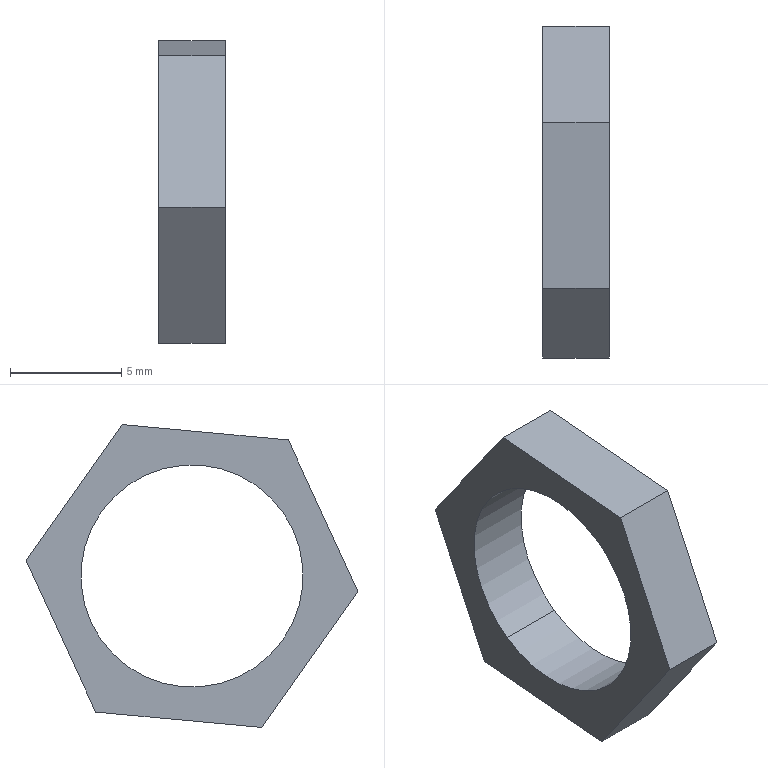Component | SolidWorks | ElectricalBoxAssembly2-1_AngleSensorComponentAssembly3-1_AngleDisplacementSensorNut-1 | 1 solid | 10 faces | box 3 x 14.95 x 13.64 mm | volume 203 mm3 | plane 8 | cylinder 2 | commonest cylinder face diameters 10 x2
STEP:
#1=COLOUR_RGB('',0.7922,0.8196,0.9333);
#2=FILL_AREA_STYLE_COLOUR('',#1);
#3=FILL_AREA_STYLE('',(#2));
#4=SURFACE_STYLE_FILL_AREA(#3);
#5=SURFACE_SIDE_STYLE('',(#4));
#6=SURFACE_STYLE_USAGE(.BOTH.,#5);
#7=PRESENTATION_STYLE_ASSIGNMENT((#6));
#8=CARTESIAN_POINT('',(33.823,8.338,68.917));
#9=VERTEX_POINT('',#8);
#10=CARTESIAN_POINT('',(33.823,8.565,68.595));
#11=VERTEX_POINT('',#10);
#12=CARTESIAN_POINT('',(33.823,8.451,68.756));
#13=DIRECTION('',(-1.,0.,0.));
#14=DIRECTION('',(0.,0.5777,-0.8163));
#15=AXIS2_PLACEMENT_3D('',#12,#13,#14);
#16=CIRCLE('',#15,0.1969);
#17=EDGE_CURVE('',#9,#11,#16,.T.);
#18=ORIENTED_EDGE('',*,*,#17,.F.);
#19=CARTESIAN_POINT('',(33.705,8.338,68.917));
#20=VERTEX_POINT('',#19);
#21=CARTESIAN_POINT('',(33.705,8.338,68.917));
#22=DIRECTION('',(-1.,0.,0.));
#23=VECTOR('',#22,39.37);
#24=LINE('',#21,#23);
#25=EDGE_CURVE('',#9,#20,#24,.T.);
#26=ORIENTED_EDGE('',*,*,#25,.T.);
#27=CARTESIAN_POINT('',(33.705,8.565,68.595));
#28=VERTEX_POINT('',#27);
#29=CARTESIAN_POINT('',(33.705,8.451,68.756));
#30=DIRECTION('',(-1.,0.,0.));
#31=DIRECTION('',(0.,0.5777,-0.8163));
#32=AXIS2_PLACEMENT_3D('',#29,#30,#31);
#33=CIRCLE('',#32,0.1969);
#34=EDGE_CURVE('',#20,#28,#33,.T.);
#35=ORIENTED_EDGE('',*,*,#34,.T.);
#36=CARTESIAN_POINT('',(33.705,8.565,68.595));
#37=DIRECTION('',(-1.,0.,0.));
#38=VECTOR('',#37,39.37);
#39=LINE('',#36,#38);
#40=EDGE_CURVE('',#11,#28,#39,.T.);
#41=ORIENTED_EDGE('',*,*,#40,.F.);
#42=EDGE_LOOP('',(#18,#26,#35,#41));
#43=FACE_OUTER_BOUND('',#42,.T.);
#44=CARTESIAN_POINT('',(33.705,8.451,68.756));
#45=DIRECTION('',(-1.,0.,0.));
#46=DIRECTION('',(0.,0.5777,-0.8163));
#47=AXIS2_PLACEMENT_3D('',#44,#45,#46);
#48=CYLINDRICAL_SURFACE('',#47,0.1969);
#49=ADVANCED_FACE('',(#43),#48,.F.);
#50=CARTESIAN_POINT('',(33.823,8.575,69.024));
#51=VERTEX_POINT('',#50);
#52=CARTESIAN_POINT('',(33.823,8.281,68.997));
#53=VERTEX_POINT('',#52);
#54=CARTESIAN_POINT('',(33.823,8.575,69.024));
#55=DIRECTION('',(-0.,-0.9957,-0.09214));
#56=VECTOR('',#55,39.37);
#57=LINE('',#54,#56);
#58=EDGE_CURVE('',#51,#53,#57,.T.);
#59=ORIENTED_EDGE('',*,*,#58,.T.);
#60=CARTESIAN_POINT('',(33.823,8.157,68.729));
#61=VERTEX_POINT('',#60);
#62=CARTESIAN_POINT('',(33.823,8.281,68.997));
#63=DIRECTION('',(-0.,-0.4181,-0.9084));
#64=VECTOR('',#63,39.37);
#65=LINE('',#62,#64);
#66=EDGE_CURVE('',#53,#61,#65,.T.);
#67=ORIENTED_EDGE('',*,*,#66,.T.);
#68=CARTESIAN_POINT('',(33.823,8.328,68.487));
#69=VERTEX_POINT('',#68);
#70=CARTESIAN_POINT('',(33.823,8.157,68.729));
#71=DIRECTION('',(-0.,0.5777,-0.8163));
#72=VECTOR('',#71,39.37);
#73=LINE('',#70,#72);
#74=EDGE_CURVE('',#61,#69,#73,.T.);
#75=ORIENTED_EDGE('',*,*,#74,.T.);
#76=CARTESIAN_POINT('',(33.823,8.622,68.515));
#77=VERTEX_POINT('',#76);
#78=CARTESIAN_POINT('',(33.823,8.328,68.487));
#79=DIRECTION('',(0.,0.9957,0.09214));
#80=VECTOR('',#79,39.37);
#81=LINE('',#78,#80);
#82=EDGE_CURVE('',#69,#77,#81,.T.);
#83=ORIENTED_EDGE('',*,*,#82,.T.);
#84=CARTESIAN_POINT('',(33.823,8.746,68.783));
#85=VERTEX_POINT('',#84);
#86=CARTESIAN_POINT('',(33.823,8.622,68.515));
#87=DIRECTION('',(0.,0.4181,0.9084));
#88=VECTOR('',#87,39.37);
#89=LINE('',#86,#88);
#90=EDGE_CURVE('',#77,#85,#89,.T.);
#91=ORIENTED_EDGE('',*,*,#90,.T.);
#92=CARTESIAN_POINT('',(33.823,8.746,68.783));
#93=DIRECTION('',(0.,-0.5777,0.8163));
#94=VECTOR('',#93,39.37);
#95=LINE('',#92,#94);
#96=EDGE_CURVE('',#85,#51,#95,.T.);
#97=ORIENTED_EDGE('',*,*,#96,.T.);
#98=EDGE_LOOP('',(#59,#67,#75,#83,#91,#97));
#99=FACE_OUTER_BOUND('',#98,.T.);
#100=CARTESIAN_POINT('',(33.823,8.451,68.756));
#101=DIRECTION('',(-1.,0.,0.));
#102=DIRECTION('',(0.,0.5777,-0.8163));
#103=AXIS2_PLACEMENT_3D('',#100,#101,#102);
#104=CIRCLE('',#103,0.1969);
#105=EDGE_CURVE('',#11,#9,#104,.T.);
#106=ORIENTED_EDGE('',*,*,#105,.T.);
#107=ORIENTED_EDGE('',*,*,#17,.T.);
#108=EDGE_LOOP('',(#106,#107));
#109=FACE_BOUND('',#108,.T.);
#110=CARTESIAN_POINT('',(33.823,8.451,68.756));
#111=DIRECTION('',(1.,-0.,-0.));
#112=DIRECTION('',(0.,-0.5777,0.8163));
#113=AXIS2_PLACEMENT_3D('',#110,#111,#112);
#114=PLANE('',#113);
#115=ADVANCED_FACE('',(#99,#109),#114,.T.);
#116=CARTESIAN_POINT('',(33.705,8.575,69.024));
#117=VERTEX_POINT('',#116);
#118=CARTESIAN_POINT('',(33.705,8.281,68.997));
#119=VERTEX_POINT('',#118);
#120=CARTESIAN_POINT('',(33.705,8.575,69.024));
#121=DIRECTION('',(-0.,-0.9957,-0.09214));
#122=VECTOR('',#121,39.37);
#123=LINE('',#120,#122);
#124=EDGE_CURVE('',#117,#119,#123,.T.);
#125=ORIENTED_EDGE('',*,*,#124,.T.);
#126=CARTESIAN_POINT('',(33.823,8.281,68.997));
#127=DIRECTION('',(-1.,0.,0.));
#128=VECTOR('',#127,39.37);
#129=LINE('',#126,#128);
#130=EDGE_CURVE('',#53,#119,#129,.T.);
#131=ORIENTED_EDGE('',*,*,#130,.F.);
#132=ORIENTED_EDGE('',*,*,#58,.F.);
#133=CARTESIAN_POINT('',(33.823,8.575,69.024));
#134=DIRECTION('',(-1.,0.,0.));
#135=VECTOR('',#134,39.37);
#136=LINE('',#133,#135);
#137=EDGE_CURVE('',#51,#117,#136,.T.);
#138=ORIENTED_EDGE('',*,*,#137,.T.);
#139=EDGE_LOOP('',(#125,#131,#132,#138));
#140=FACE_OUTER_BOUND('',#139,.T.);
#141=CARTESIAN_POINT('',(33.823,8.575,69.024));
#142=DIRECTION('',(-0.,0.09214,-0.9957));
#143=DIRECTION('',(0.,0.9957,0.09214));
#144=AXIS2_PLACEMENT_3D('',#141,#142,#143);
#145=PLANE('',#144);
#146=ADVANCED_FACE('',(#140),#145,.F.);
#147=CARTESIAN_POINT('',(33.705,8.157,68.729));
#148=VERTEX_POINT('',#147);
#149=CARTESIAN_POINT('',(33.705,8.281,68.997));
#150=DIRECTION('',(-0.,-0.4181,-0.9084));
#151=VECTOR('',#150,39.37);
#152=LINE('',#149,#151);
#153=EDGE_CURVE('',#119,#148,#152,.T.);
#154=ORIENTED_EDGE('',*,*,#153,.T.);
#155=CARTESIAN_POINT('',(33.823,8.157,68.729));
#156=DIRECTION('',(-1.,0.,0.));
#157=VECTOR('',#156,39.37);
#158=LINE('',#155,#157);
#159=EDGE_CURVE('',#61,#148,#158,.T.);
#160=ORIENTED_EDGE('',*,*,#159,.F.);
#161=ORIENTED_EDGE('',*,*,#66,.F.);
#162=ORIENTED_EDGE('',*,*,#130,.T.);
#163=EDGE_LOOP('',(#154,#160,#161,#162));
#164=FACE_OUTER_BOUND('',#163,.T.);
#165=CARTESIAN_POINT('',(33.823,8.281,68.997));
#166=DIRECTION('',(-0.,0.9084,-0.4181));
#167=DIRECTION('',(0.,0.4181,0.9084));
#168=AXIS2_PLACEMENT_3D('',#165,#166,#167);
#169=PLANE('',#168);
#170=ADVANCED_FACE('',(#164),#169,.F.);
#171=CARTESIAN_POINT('',(33.705,8.328,68.487));
#172=VERTEX_POINT('',#171);
#173=CARTESIAN_POINT('',(33.705,8.157,68.729));
#174=DIRECTION('',(-0.,0.5777,-0.8163));
#175=VECTOR('',#174,39.37);
#176=LINE('',#173,#175);
#177=EDGE_CURVE('',#148,#172,#176,.T.);
#178=ORIENTED_EDGE('',*,*,#177,.T.);
#179=CARTESIAN_POINT('',(33.823,8.328,68.487));
#180=DIRECTION('',(-1.,0.,0.));
#181=VECTOR('',#180,39.37);
#182=LINE('',#179,#181);
#183=EDGE_CURVE('',#69,#172,#182,.T.);
#184=ORIENTED_EDGE('',*,*,#183,.F.);
#185=ORIENTED_EDGE('',*,*,#74,.F.);
#186=ORIENTED_EDGE('',*,*,#159,.T.);
#187=EDGE_LOOP('',(#178,#184,#185,#186));
#188=FACE_OUTER_BOUND('',#187,.T.);
#189=CARTESIAN_POINT('',(33.823,8.157,68.729));
#190=DIRECTION('',(0.,0.8163,0.5777));
#191=DIRECTION('',(0.,-0.5777,0.8163));
#192=AXIS2_PLACEMENT_3D('',#189,#190,#191);
#193=PLANE('',#192);
#194=ADVANCED_FACE('',(#188),#193,.F.);
#195=CARTESIAN_POINT('',(33.705,8.622,68.515));
#196=VERTEX_POINT('',#195);
#197=CARTESIAN_POINT('',(33.705,8.328,68.487));
#198=DIRECTION('',(0.,0.9957,0.09214));
#199=VECTOR('',#198,39.37);
#200=LINE('',#197,#199);
#201=EDGE_CURVE('',#172,#196,#200,.T.);
#202=ORIENTED_EDGE('',*,*,#201,.T.);
#203=CARTESIAN_POINT('',(33.823,8.622,68.515));
#204=DIRECTION('',(-1.,0.,0.));
#205=VECTOR('',#204,39.37);
#206=LINE('',#203,#205);
#207=EDGE_CURVE('',#77,#196,#206,.T.);
#208=ORIENTED_EDGE('',*,*,#207,.F.);
#209=ORIENTED_EDGE('',*,*,#82,.F.);
#210=ORIENTED_EDGE('',*,*,#183,.T.);
#211=EDGE_LOOP('',(#202,#208,#209,#210));
#212=FACE_OUTER_BOUND('',#211,.T.);
#213=CARTESIAN_POINT('',(33.823,8.328,68.487));
#214=DIRECTION('',(0.,-0.09214,0.9957));
#215=DIRECTION('',(-0.,-0.9957,-0.09214));
#216=AXIS2_PLACEMENT_3D('',#213,#214,#215);
#217=PLANE('',#216);
#218=ADVANCED_FACE('',(#212),#217,.F.);
#219=CARTESIAN_POINT('',(33.705,8.746,68.783));
#220=VERTEX_POINT('',#219);
#221=CARTESIAN_POINT('',(33.705,8.622,68.515));
#222=DIRECTION('',(0.,0.4181,0.9084));
#223=VECTOR('',#222,39.37);
#224=LINE('',#221,#223);
#225=EDGE_CURVE('',#196,#220,#224,.T.);
#226=ORIENTED_EDGE('',*,*,#225,.T.);
#227=CARTESIAN_POINT('',(33.823,8.746,68.783));
#228=DIRECTION('',(-1.,0.,0.));
#229=VECTOR('',#228,39.37);
#230=LINE('',#227,#229);
#231=EDGE_CURVE('',#85,#220,#230,.T.);
#232=ORIENTED_EDGE('',*,*,#231,.F.);
#233=ORIENTED_EDGE('',*,*,#90,.F.);
#234=ORIENTED_EDGE('',*,*,#207,.T.);
#235=EDGE_LOOP('',(#226,#232,#233,#234));
#236=FACE_OUTER_BOUND('',#235,.T.);
#237=CARTESIAN_POINT('',(33.823,8.622,68.515));
#238=DIRECTION('',(0.,-0.9084,0.4181));
#239=DIRECTION('',(-0.,-0.4181,-0.9084));
#240=AXIS2_PLACEMENT_3D('',#237,#238,#239);
#241=PLANE('',#240);
#242=ADVANCED_FACE('',(#236),#241,.F.);
#243=CARTESIAN_POINT('',(33.705,8.746,68.783));
#244=DIRECTION('',(0.,-0.5777,0.8163));
#245=VECTOR('',#244,39.37);
#246=LINE('',#243,#245);
#247=EDGE_CURVE('',#220,#117,#246,.T.);
#248=ORIENTED_EDGE('',*,*,#247,.T.);
#249=ORIENTED_EDGE('',*,*,#137,.F.);
#250=ORIENTED_EDGE('',*,*,#96,.F.);
#251=ORIENTED_EDGE('',*,*,#231,.T.);
#252=EDGE_LOOP('',(#248,#249,#250,#251));
#253=FACE_OUTER_BOUND('',#252,.T.);
#254=CARTESIAN_POINT('',(33.823,8.746,68.783));
#255=DIRECTION('',(-0.,-0.8163,-0.5777));
#256=DIRECTION('',(-0.,0.5777,-0.8163));
#257=AXIS2_PLACEMENT_3D('',#254,#255,#256);
#258=PLANE('',#257);
#259=ADVANCED_FACE('',(#253),#258,.F.);
#260=CARTESIAN_POINT('',(33.705,8.451,68.756));
#261=DIRECTION('',(-1.,0.,0.));
#262=DIRECTION('',(0.,0.5777,-0.8163));
#263=AXIS2_PLACEMENT_3D('',#260,#261,#262);
#264=CIRCLE('',#263,0.1969);
#265=EDGE_CURVE('',#28,#20,#264,.T.);
#266=ORIENTED_EDGE('',*,*,#265,.F.);
#267=ORIENTED_EDGE('',*,*,#34,.F.);
#268=EDGE_LOOP('',(#266,#267));
#269=FACE_BOUND('',#268,.T.);
#270=ORIENTED_EDGE('',*,*,#124,.F.);
#271=ORIENTED_EDGE('',*,*,#247,.F.);
#272=ORIENTED_EDGE('',*,*,#225,.F.);
#273=ORIENTED_EDGE('',*,*,#201,.F.);
#274=ORIENTED_EDGE('',*,*,#177,.F.);
#275=ORIENTED_EDGE('',*,*,#153,.F.);
#276=EDGE_LOOP('',(#270,#271,#272,#273,#274,#275));
#277=FACE_OUTER_BOUND('',#276,.T.);
#278=CARTESIAN_POINT('',(33.705,8.451,68.756));
#279=DIRECTION('',(1.,-0.,-0.));
#280=DIRECTION('',(0.,-0.5777,0.8163));
#281=AXIS2_PLACEMENT_3D('',#278,#279,#280);
#282=PLANE('',#281);
#283=ADVANCED_FACE('',(#269,#277),#282,.F.);
#284=ORIENTED_EDGE('',*,*,#25,.F.);
#285=ORIENTED_EDGE('',*,*,#105,.F.);
#286=ORIENTED_EDGE('',*,*,#40,.T.);
#287=ORIENTED_EDGE('',*,*,#265,.T.);
#288=EDGE_LOOP('',(#284,#285,#286,#287));
#289=FACE_OUTER_BOUND('',#288,.T.);
#290=CARTESIAN_POINT('',(33.705,8.451,68.756));
#291=DIRECTION('',(-1.,0.,0.));
#292=DIRECTION('',(0.,0.5777,-0.8163));
#293=AXIS2_PLACEMENT_3D('',#290,#291,#292);
#294=CYLINDRICAL_SURFACE('',#293,0.1969);
#295=ADVANCED_FACE('',(#289),#294,.F.);
#296=CLOSED_SHELL('',(#49,#115,#146,#170,#194,#218,#242,#259,#283,#295));
#297=MANIFOLD_SOLID_BREP('',#296);
#298=STYLED_ITEM('',(#7),#297);
#299=PRESENTATION_LAYER_ASSIGNMENT('','',(#298));
#300=(LENGTH_UNIT()NAMED_UNIT(*)SI_UNIT($,.METRE.));
#301=LENGTH_MEASURE_WITH_UNIT(LENGTH_MEASURE(0.0254),#300);
#302=DIMENSIONAL_EXPONENTS(1.,0.,0.,0.,0.,0.,0.);
#303=(CONVERSION_BASED_UNIT('',#301)LENGTH_UNIT()NAMED_UNIT(#302));
#304=UNCERTAINTY_MEASURE_WITH_UNIT(LENGTH_MEASURE(0.00001),#303,'','');
#305=(NAMED_UNIT(*)PLANE_ANGLE_UNIT()SI_UNIT($,.RADIAN.));
#306=(NAMED_UNIT(*)SI_UNIT($,.STERADIAN.)SOLID_ANGLE_UNIT());
#307=(GEOMETRIC_REPRESENTATION_CONTEXT(3)GLOBAL_UNCERTAINTY_ASSIGNED_CONTEXT((#304))GLOBAL_UNIT_ASSIGNED_CONTEXT((#303,#305,#306))REPRESENTATION_CONTEXT('',''));
#308=MECHANICAL_DESIGN_GEOMETRIC_PRESENTATION_REPRESENTATION('',(#298),#307);
#309=CARTESIAN_POINT('',(0.,0.,0.));
#310=DIRECTION('',(0.,0.,1.));
#311=DIRECTION('',(1.,0.,0.));
#312=AXIS2_PLACEMENT_3D('',#309,#310,#311);
#313=(LENGTH_UNIT()NAMED_UNIT(*)SI_UNIT($,.METRE.));
#314=LENGTH_MEASURE_WITH_UNIT(LENGTH_MEASURE(0.0254),#313);
#315=DIMENSIONAL_EXPONENTS(1.,0.,0.,0.,0.,0.,0.);
#316=(CONVERSION_BASED_UNIT('',#314)LENGTH_UNIT()NAMED_UNIT(#315));
#317=UNCERTAINTY_MEASURE_WITH_UNIT(LENGTH_MEASURE(0.00001),#316,'','');
#318=(NAMED_UNIT(*)PLANE_ANGLE_UNIT()SI_UNIT($,.RADIAN.));
#319=(NAMED_UNIT(*)SI_UNIT($,.STERADIAN.)SOLID_ANGLE_UNIT());
#320=(GEOMETRIC_REPRESENTATION_CONTEXT(3)GLOBAL_UNCERTAINTY_ASSIGNED_CONTEXT((#317))GLOBAL_UNIT_ASSIGNED_CONTEXT((#316,#318,#319))REPRESENTATION_CONTEXT('',''));
#321=ADVANCED_BREP_SHAPE_REPRESENTATION('',(#297,#312),#320);